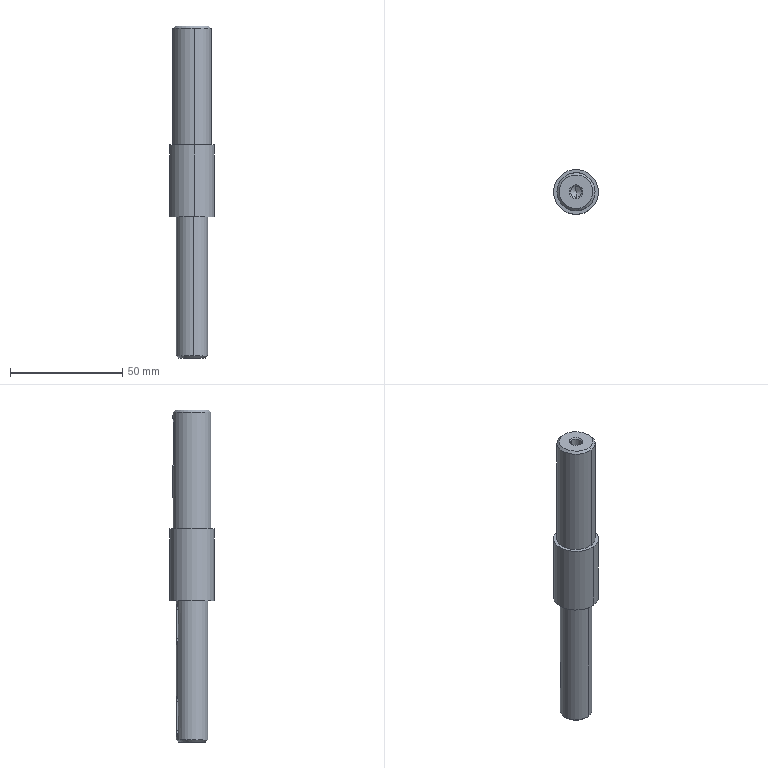Component | SolidWorks | ConnectionAxis-1 | 1 solid | 44 faces | box 20 x 20 x 148 mm | volume 30101 mm3 | cylinder 19 | plane 13 | cone 12 | commonest cylinder face diameters 5 x13 17 x2 14 x2 20 x2
build123d program:
from build123d import *

# Parameters (mm, degrees)
SKETCH1_W                          = 32
SKETCH1_H                          = 10
SKETCH2_R                          = 7
BOSS_EXTRUDE1_DEPTH                = 62
SKETCH3_R                          = 7
BOSS_EXTRUDE2_DEPTH                = 1
BOSS_EXTRUDE2_TAPER                = 45
SKETCH4_R                          = 8.5
BOSS_EXTRUDE3_DEPTH                = 52
SKETCH5_R                          = 8.5
BOSS_EXTRUDE4_DEPTH                = 1
BOSS_EXTRUDE4_TAPER                = 45
CUT_EXTRUDE1_REACH                 = 77.974
CUT_EXTRUDE1_END_RADIUS            = 7
CUT_EXTRUDE2_REACH                 = 77.974
CUT_EXTRUDE2_END_RADIUS            = 7
CUT_EXTRUDE3_REACH                 = 77.974
CUT_EXTRUDE3_END_RADIUS            = 8.5
F_5_0_5_DIAMETER_HOLE1_D           = 5
F_5_0_5_DIAMETER_HOLE1_DEPTH       = 17
F_5_0_5_DIAMETER_HOLE1_CSINK_D     = 6.05
F_5_0_5_DIAMETER_HOLE1_CSINK_ANGLE = 90
F_5_0_5_DIAMETER_HOLE1_TIP         = 1.502
F_5_0_5_DIAMETER_HOLE2_D           = 5
F_5_0_5_DIAMETER_HOLE2_DEPTH       = 17
F_5_0_5_DIAMETER_HOLE2_CSINK_D     = 6.05
F_5_0_5_DIAMETER_HOLE2_CSINK_ANGLE = 90
F_5_0_5_DIAMETER_HOLE2_TIP         = 1.502


with BuildPart() as part:
    # Sketch1 → Revolve1 (revolve)
    with BuildSketch(Plane(origin=(0, 0, 0), x_dir=(-1, 0, 0), z_dir=(0, 0, -1)), mode=Mode.PRIVATE) as revolve1_sk:
        with Locations((-5, 5)):
            Rectangle(SKETCH1_W, SKETCH1_H)
    revolve(revolve1_sk.sketch.rotate(Axis((21, 0, 0), (-1, 0, 0)), 270), axis=Axis((21, 0, 0), (-1, 0, 0)))

    # Sketch2 → Boss-Extrude1 (add)
    with BuildSketch(Plane.ZY.offset(11)):
        Circle(SKETCH2_R)
    extrude(amount=BOSS_EXTRUDE1_DEPTH)

    # Sketch3 → Boss-Extrude2 (add)
    with BuildSketch(Plane.ZY.offset(73)):
        Circle(SKETCH3_R)
    extrude(amount=BOSS_EXTRUDE2_DEPTH, taper=BOSS_EXTRUDE2_TAPER)

    # Sketch4 → Boss-Extrude3 (add)
    with BuildSketch(Plane(origin=(21, 0, 0), x_dir=(0, 0, -1), z_dir=(1, 0, 0))):
        Circle(SKETCH4_R)
    extrude(amount=BOSS_EXTRUDE3_DEPTH)

    # Sketch5 → Boss-Extrude4 (add)
    with BuildSketch(Plane(origin=(73, 0, 0), x_dir=(0, 0, -1), z_dir=(1, 0, 0))):
        Circle(SKETCH5_R)
    extrude(amount=BOSS_EXTRUDE4_DEPTH, taper=BOSS_EXTRUDE4_TAPER)

    # Cut-Extrude1: up to this cylinder (the profile starts inside it)
    cut_extrude1_end = Plane(origin=(-62.5, 0, 0), z_dir=(1, 0, 0)) * Cylinder(CUT_EXTRUDE1_END_RADIUS, 170.948, mode=Mode.PRIVATE)
    # Sketch6 → Cut-Extrude1 (cut, up to the surface)
    with BuildSketch(Plane(origin=(0, 0, 4), x_dir=(-1, 0, 0), z_dir=(0, 0, -1)), mode=Mode.PRIVATE) as cut_extrude1_sk1:
        with BuildLine():
            Line((69, 2.5), (56, 2.5))
            ThreePointArc((56, 2.5), (53.5, 0), (56, -2.5))
            Line((56, -2.5), (69, -2.5))
            ThreePointArc((69, -2.5), (71.5, 0), (69, 2.5))
        make_face()
    cut_extrude1_tool1 = extrude(cut_extrude1_sk1.sketch, amount=-CUT_EXTRUDE1_REACH, mode=Mode.PRIVATE) & cut_extrude1_end
    add(cut_extrude1_tool1.solids().sort_by_distance((-62.5, 0, 4))[0], mode=Mode.SUBTRACT)

    # Cut-Extrude2: up to this cylinder (the profile starts inside it)
    cut_extrude2_end = Plane(origin=(-21.5, 0, 0), z_dir=(1, 0, 0)) * Cylinder(CUT_EXTRUDE2_END_RADIUS, 170.948, mode=Mode.PRIVATE)
    # Sketch7 → Cut-Extrude2 (cut, up to the surface)
    with BuildSketch(Plane(origin=(0, 0, 4), x_dir=(-1, 0, 0), z_dir=(0, 0, -1)), mode=Mode.PRIVATE) as cut_extrude2_sk1:
        with BuildLine():
            Line((28, 2.5), (15, 2.5))
            ThreePointArc((15, 2.5), (12.5, 0), (15, -2.5))
            Line((15, -2.5), (28, -2.5))
            ThreePointArc((28, -2.5), (30.5, 0), (28, 2.5))
        make_face()
    cut_extrude2_tool1 = extrude(cut_extrude2_sk1.sketch, amount=-CUT_EXTRUDE2_REACH, mode=Mode.PRIVATE) & cut_extrude2_end
    add(cut_extrude2_tool1.solids().sort_by_distance((-21.5, 0, 4))[0], mode=Mode.SUBTRACT)

    # Cut-Extrude3: up to this cylinder (the profile starts inside it)
    cut_extrude3_end = Plane(origin=(59.5, 0, 0), z_dir=(-1, 0, 0)) * Cylinder(CUT_EXTRUDE3_END_RADIUS, 173.948, mode=Mode.PRIVATE)
    # Sketch8 → Cut-Extrude3 (cut, up to the surface)
    with BuildSketch(Plane(origin=(0, 0, 4), x_dir=(-1, 0, 0), z_dir=(0, 0, -1)), mode=Mode.PRIVATE) as cut_extrude3_sk1:
        with BuildLine():
            Line((-51, 2.5), (-68, 2.5))
            ThreePointArc((-68, 2.5), (-70.5, 0), (-68, -2.5))
            Line((-68, -2.5), (-51, -2.5))
            ThreePointArc((-51, -2.5), (-48.5, 0), (-51, 2.5))
        make_face()
    cut_extrude3_tool1 = extrude(cut_extrude3_sk1.sketch, amount=-CUT_EXTRUDE3_REACH, mode=Mode.PRIVATE) & cut_extrude3_end
    add(cut_extrude3_tool1.solids().sort_by_distance((59.5, 0, 4))[0], mode=Mode.SUBTRACT)

    # 5.0 _5_ Diameter Hole1
    with Locations(Plane(origin=(74, 0, 0), x_dir=(0, 0, -1), z_dir=(1, 0, 0))):
        with Locations((0, 0)):
            CounterSinkHole(F_5_0_5_DIAMETER_HOLE1_D / 2, F_5_0_5_DIAMETER_HOLE1_CSINK_D / 2, depth=F_5_0_5_DIAMETER_HOLE1_DEPTH, counter_sink_angle=F_5_0_5_DIAMETER_HOLE1_CSINK_ANGLE)
            with Locations((0, 0, -(F_5_0_5_DIAMETER_HOLE1_DEPTH + F_5_0_5_DIAMETER_HOLE1_TIP / 2))):  # 118° drill point
                Cone(0, F_5_0_5_DIAMETER_HOLE1_D / 2, F_5_0_5_DIAMETER_HOLE1_TIP, mode=Mode.SUBTRACT)

    # 5.0 _5_ Diameter Hole2
    with Locations(Plane.ZY.offset(74)):
        with Locations((0, 0)):
            CounterSinkHole(F_5_0_5_DIAMETER_HOLE2_D / 2, F_5_0_5_DIAMETER_HOLE2_CSINK_D / 2, depth=F_5_0_5_DIAMETER_HOLE2_DEPTH, counter_sink_angle=F_5_0_5_DIAMETER_HOLE2_CSINK_ANGLE)
            with Locations((0, 0, -(F_5_0_5_DIAMETER_HOLE2_DEPTH + F_5_0_5_DIAMETER_HOLE2_TIP / 2))):  # 118° drill point
                Cone(0, F_5_0_5_DIAMETER_HOLE2_D / 2, F_5_0_5_DIAMETER_HOLE2_TIP, mode=Mode.SUBTRACT)


solid = part.part

# Placed as in the assembly
solid = solid.moved(Location((-329.5, -291, -300.769), (-90, -7.062, -90)))